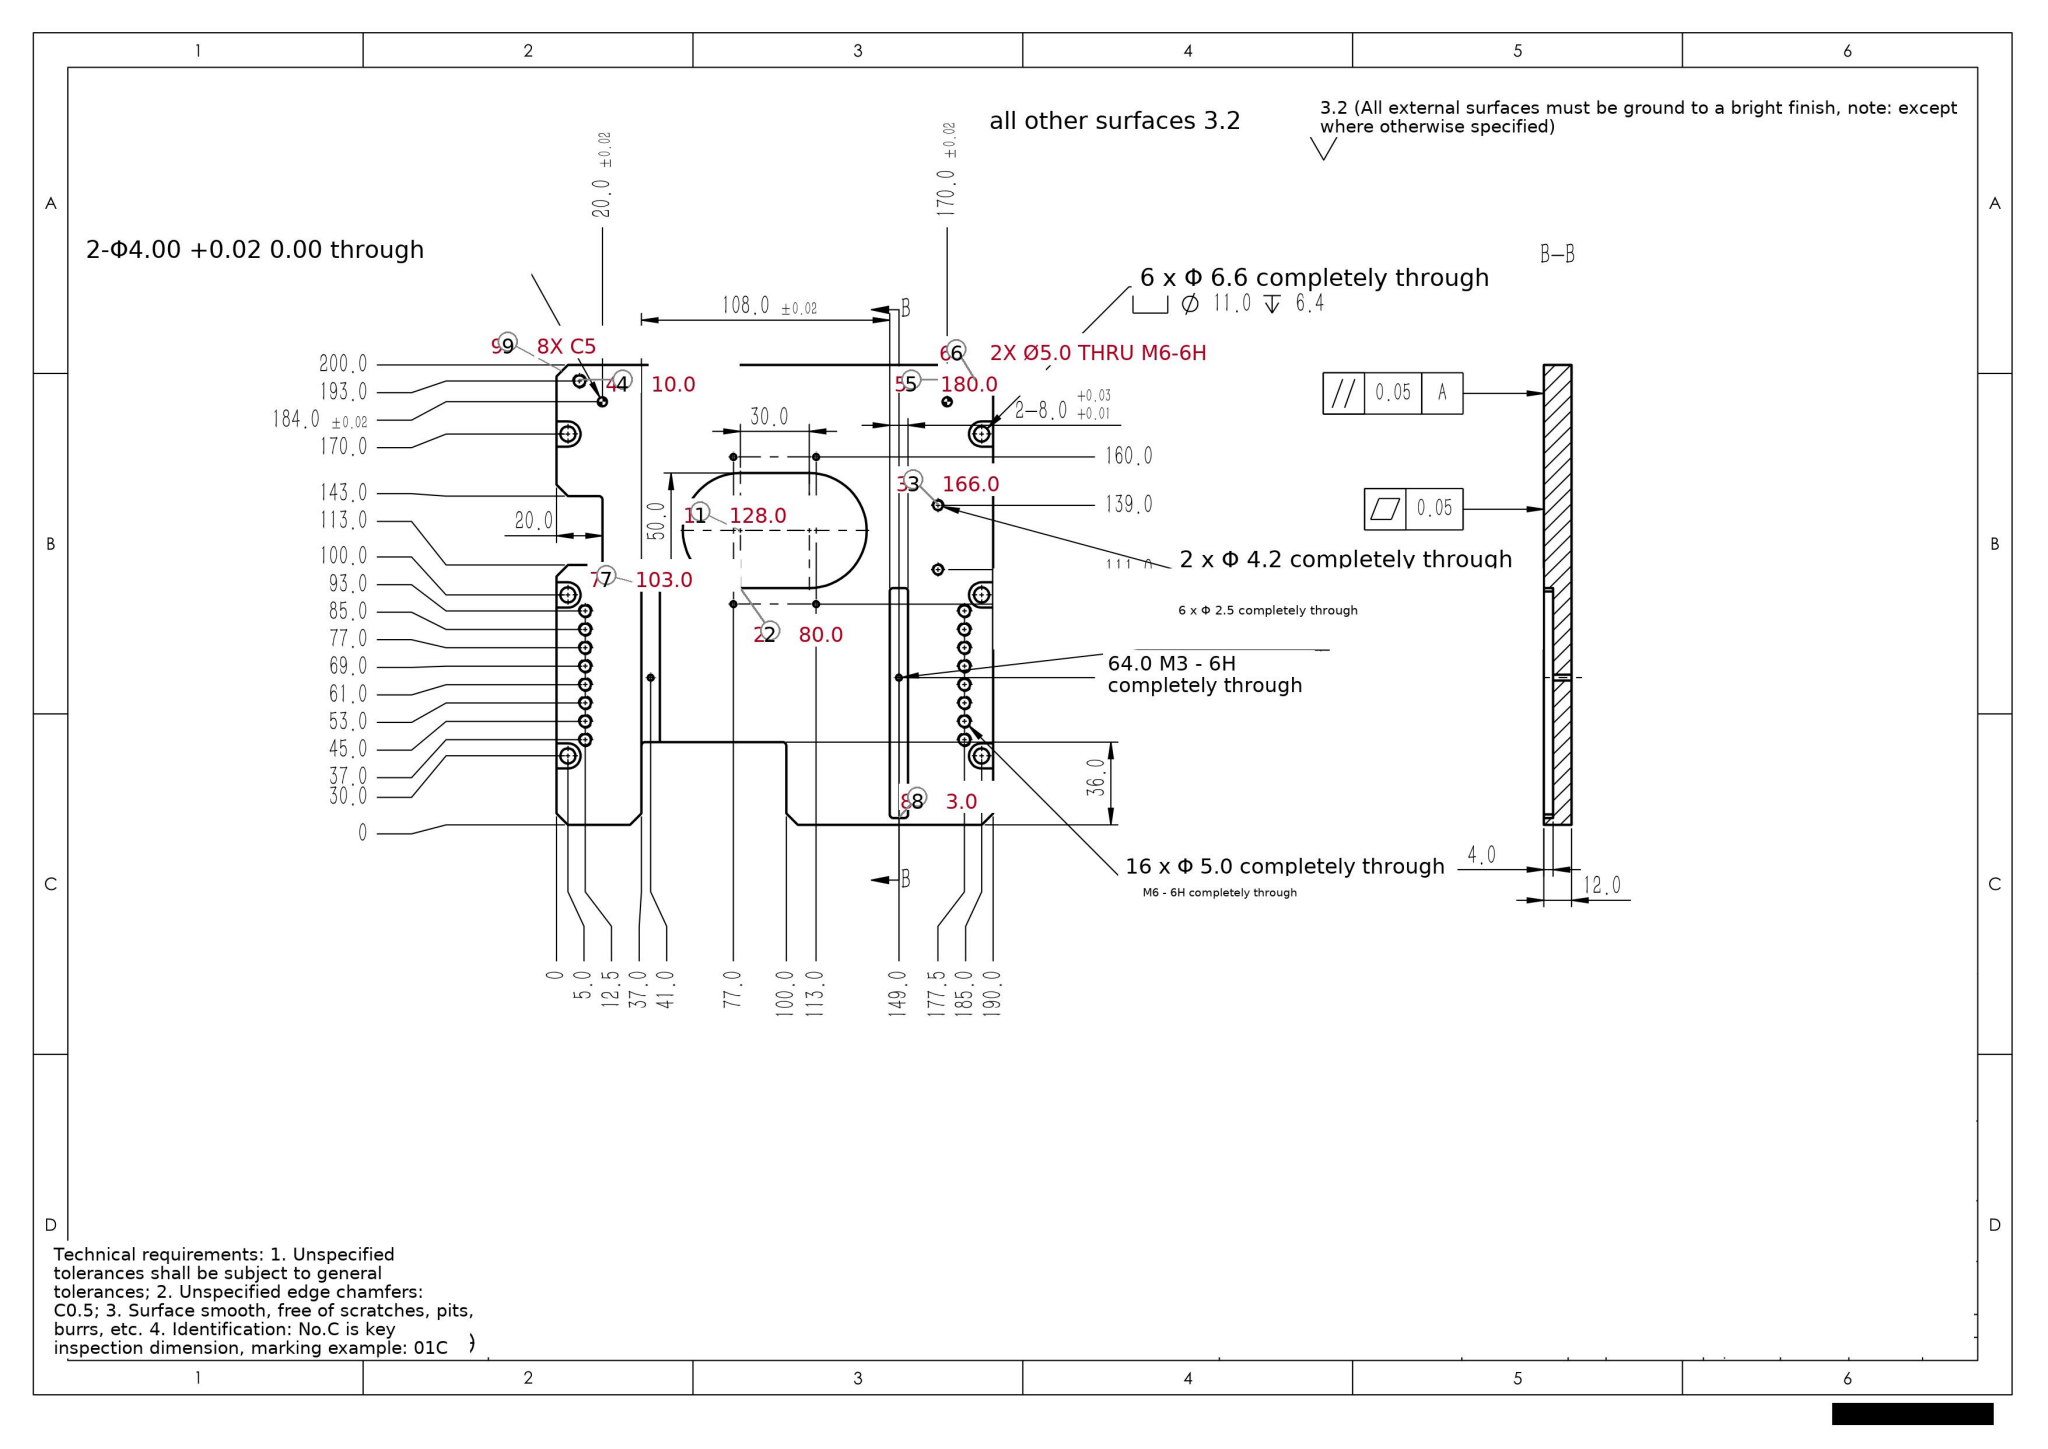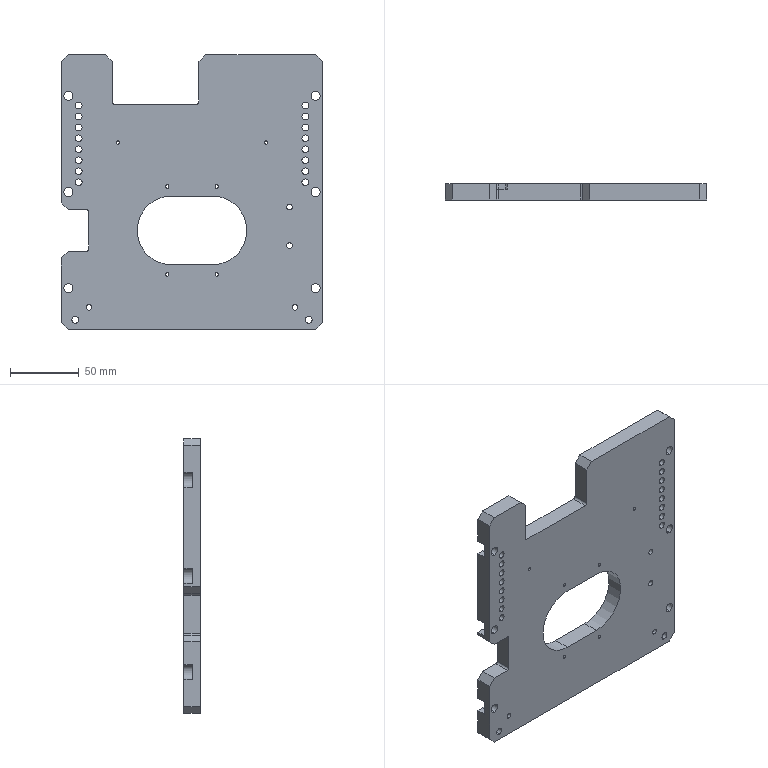Part | SolidWorks | mm | 1 solid | 136 faces | box 190 x 12 x 200 mm | volume 363235 mm3 | cylinder 86 | plane 50 | commonest cylinder face diameters 5 x36 6.6 x12 2.5 x12 3 x10 11 x6 4.2 x4 4 x4 50 x2
build123d program:
from build123d import *

# Parameters (mm, degrees)
SKETCH1_W                                       = 190
SKETCH1_H                                       = 200
BOSS_EXTRUDE1_DEPTH                             = 6
M6_TAPPED_HOLE1_D                               = 5
SKETCH4_W                                       = 8
SKETCH4_H                                       = 100
CUT_EXTRUDE1_DEPTH                              = 4
SIZE_MM_DOWEL_PIN_HOLE_0_D                      = 4
M6_TAPPED_HOLE2_D                               = 5
LPATTERN1_COUNT                                 = 8
LPATTERN1_PITCH                                 = 8
SKETCH14_W                                      = 63
SKETCH14_H                                      = 36
SKETCH14_W_2                                    = 20
SKETCH14_H_2                                    = 30
CUT_EXTRUDE3_DEPTH                              = 139.452
M3_TAPPED_HOLE1_D                               = 2.5
M6_HEX_SOCKET_HEAD_CAP_SCREW_CBORE1_D           = 6.6
M6_HEX_SOCKET_HEAD_CAP_SCREW_CBORE1_CBORE_D     = 11
M6_HEX_SOCKET_HEAD_CAP_SCREW_CBORE1_CBORE_DEPTH = 6.4
SKETCH13_W                                      = 5
SKETCH13_H                                      = 11
CUT_EXTRUDE2_DEPTH                              = 6.4
CHAMFER1_SIZE                                   = 5
FILLET1_R                                       = 1.5
M5_TAPPED_HOLE1_D                               = 4.2


with BuildPart() as part:
    # Sketch1 → Boss-Extrude1 (new, symmetric)
    with BuildSketch(Plane(origin=(0, 0, 0), x_dir=(1, 0, 0), z_dir=(0, 1, 0))):
        Rectangle(SKETCH1_W, SKETCH1_H)
    extrude(amount=BOSS_EXTRUDE1_DEPTH, both=True)

    # M6 Tapped Hole1 (through all)
    with Locations(Plane(origin=(0, 6, 0), x_dir=(1, 0, 0), z_dir=(0, 1, 0))):
        with Locations((85, 93), (-85, 93)):
            Hole(M6_TAPPED_HOLE1_D / 2)

    # Sketch4 → Cut-Extrude1 (cut)
    with BuildSketch(Plane(origin=(0, 6, 0), x_dir=(1, 0, 0), z_dir=(0, 1, 0))):
        with Locations((-54, -47)):
            Rectangle(SKETCH4_W, SKETCH4_H)
        with Locations((54, -47)):
            Rectangle(SKETCH4_W, SKETCH4_H)
    extrude(amount=-CUT_EXTRUDE1_DEPTH, mode=Mode.SUBTRACT)

    # Size mm Dowel Pin Hole 0 (through all)
    with Locations(Plane(origin=(0, 6, 0), x_dir=(1, 0, 0), z_dir=(0, 1, 0))):
        with Locations((-75, 84), (75, 84)):
            Hole(SIZE_MM_DOWEL_PIN_HOLE_0_D / 2)

    # M6 Tapped Hole2 (through all)
    with Locations(Plane(origin=(0, 6, 0), x_dir=(1, 0, 0), z_dir=(0, 1, 0))):
        with Locations((-82.5, -7), (82.5, -7)):
            m6_tapped_hole2 = Hole(M6_TAPPED_HOLE2_D / 2)

    # LPattern1: M6 Tapped Hole2 ×8
    with Locations(*[(0, 0, i * LPATTERN1_PITCH) for i in range(1, LPATTERN1_COUNT)]):
        add(m6_tapped_hole2, mode=Mode.SUBTRACT)

    # Sketch14 → Cut-Extrude3 (cut, through all)
    with BuildSketch(Plane(origin=(0, 6, 0), x_dir=(1, 0, 0), z_dir=(0, 1, 0))):
        with BuildLine():
            Line((-15, 53), (15, 53))
            ThreePointArc((15, 53), (40, 28), (15, 3))
            Line((15, 3), (-15, 3))
            ThreePointArc((-15, 3), (-40, 28), (-15, 53))
        make_face()
        with Locations((-26.5, -82)):
            Rectangle(SKETCH14_W, SKETCH14_H)
        with Locations((-85, 28)):
            Rectangle(SKETCH14_W_2, SKETCH14_H_2)
    extrude(amount=-CUT_EXTRUDE3_DEPTH, mode=Mode.SUBTRACT)

    # M3 Tapped Hole1 (through all)
    with Locations(Plane(origin=(0, 6, 0), x_dir=(1, 0, 0), z_dir=(0, 1, 0))):
        with Locations((-54, -36), (54, -36), (18, -4), (-18, -4), (18, 60), (-18, 60)):
            Hole(M3_TAPPED_HOLE1_D / 2)

    # M6 Hex Socket Head Cap Screw CBORE1 (through all)
    with Locations(Plane(origin=(0, 6, 0), x_dir=(1, 0, 0), z_dir=(0, 1, 0))):
        with Locations((-90, 70), (90, 70), (-90, 0), (-90, -70), (90, 0), (90, -70)):
            CounterBoreHole(M6_HEX_SOCKET_HEAD_CAP_SCREW_CBORE1_D / 2, M6_HEX_SOCKET_HEAD_CAP_SCREW_CBORE1_CBORE_D / 2, M6_HEX_SOCKET_HEAD_CAP_SCREW_CBORE1_CBORE_DEPTH)

    # Sketch13 → Cut-Extrude2 (cut)
    with BuildSketch(Plane(origin=(0, 6, 0), x_dir=(1, 0, 0), z_dir=(0, 1, 0))):
        with Locations((-92.5, 70)):
            Rectangle(SKETCH13_W, SKETCH13_H)
        with Locations((-92.5, 0)):
            Rectangle(SKETCH13_W, SKETCH13_H)
        with Locations((-92.5, -70)):
            Rectangle(SKETCH13_W, SKETCH13_H)
        with Locations((92.5, 70)):
            Rectangle(SKETCH13_W, SKETCH13_H)
        with Locations((92.5, 0)):
            Rectangle(SKETCH13_W, SKETCH13_H)
        with Locations((92.5, -70)):
            Rectangle(SKETCH13_W, SKETCH13_H)
    extrude(amount=-CUT_EXTRUDE2_DEPTH, mode=Mode.SUBTRACT)

    # Chamfer1
    chamfer1_edges = [part.edges().sort_by_distance(p)[0] for p in [
        (-58, 0, 100),
        (5, 0, 100),
        (-95, 0, -13),
        (-95, 0, -43),
        (95, 0, 100),
        (-95, 0, 100),
        (-95, 0, -100),
        (95, 0, -100),
    ]]
    chamfer(chamfer1_edges, length=CHAMFER1_SIZE)

    # Fillet1
    fillet1_edges = [part.edges().sort_by_distance(p)[0] for p in [
        (-58, -2, 64),
        (5, 0, 64),
        (-75, 0, -43),
        (-75, 0, -13),
        (-58, 4, -3),
        (-50, 4, -3),
        (50, 4, -3),
        (58, 4, -3),
        (58, 4, 97),
        (50, 4, 97),
    ]]
    fillet(fillet1_edges, radius=FILLET1_R)

    # M5 Tapped Hole1 (through all)
    with Locations(Plane(origin=(0, 6, 0), x_dir=(1, 0, 0), z_dir=(0, 1, 0))):
        with Locations((71, 11), (71, 39)):
            Hole(M5_TAPPED_HOLE1_D / 2)


solid = part.part